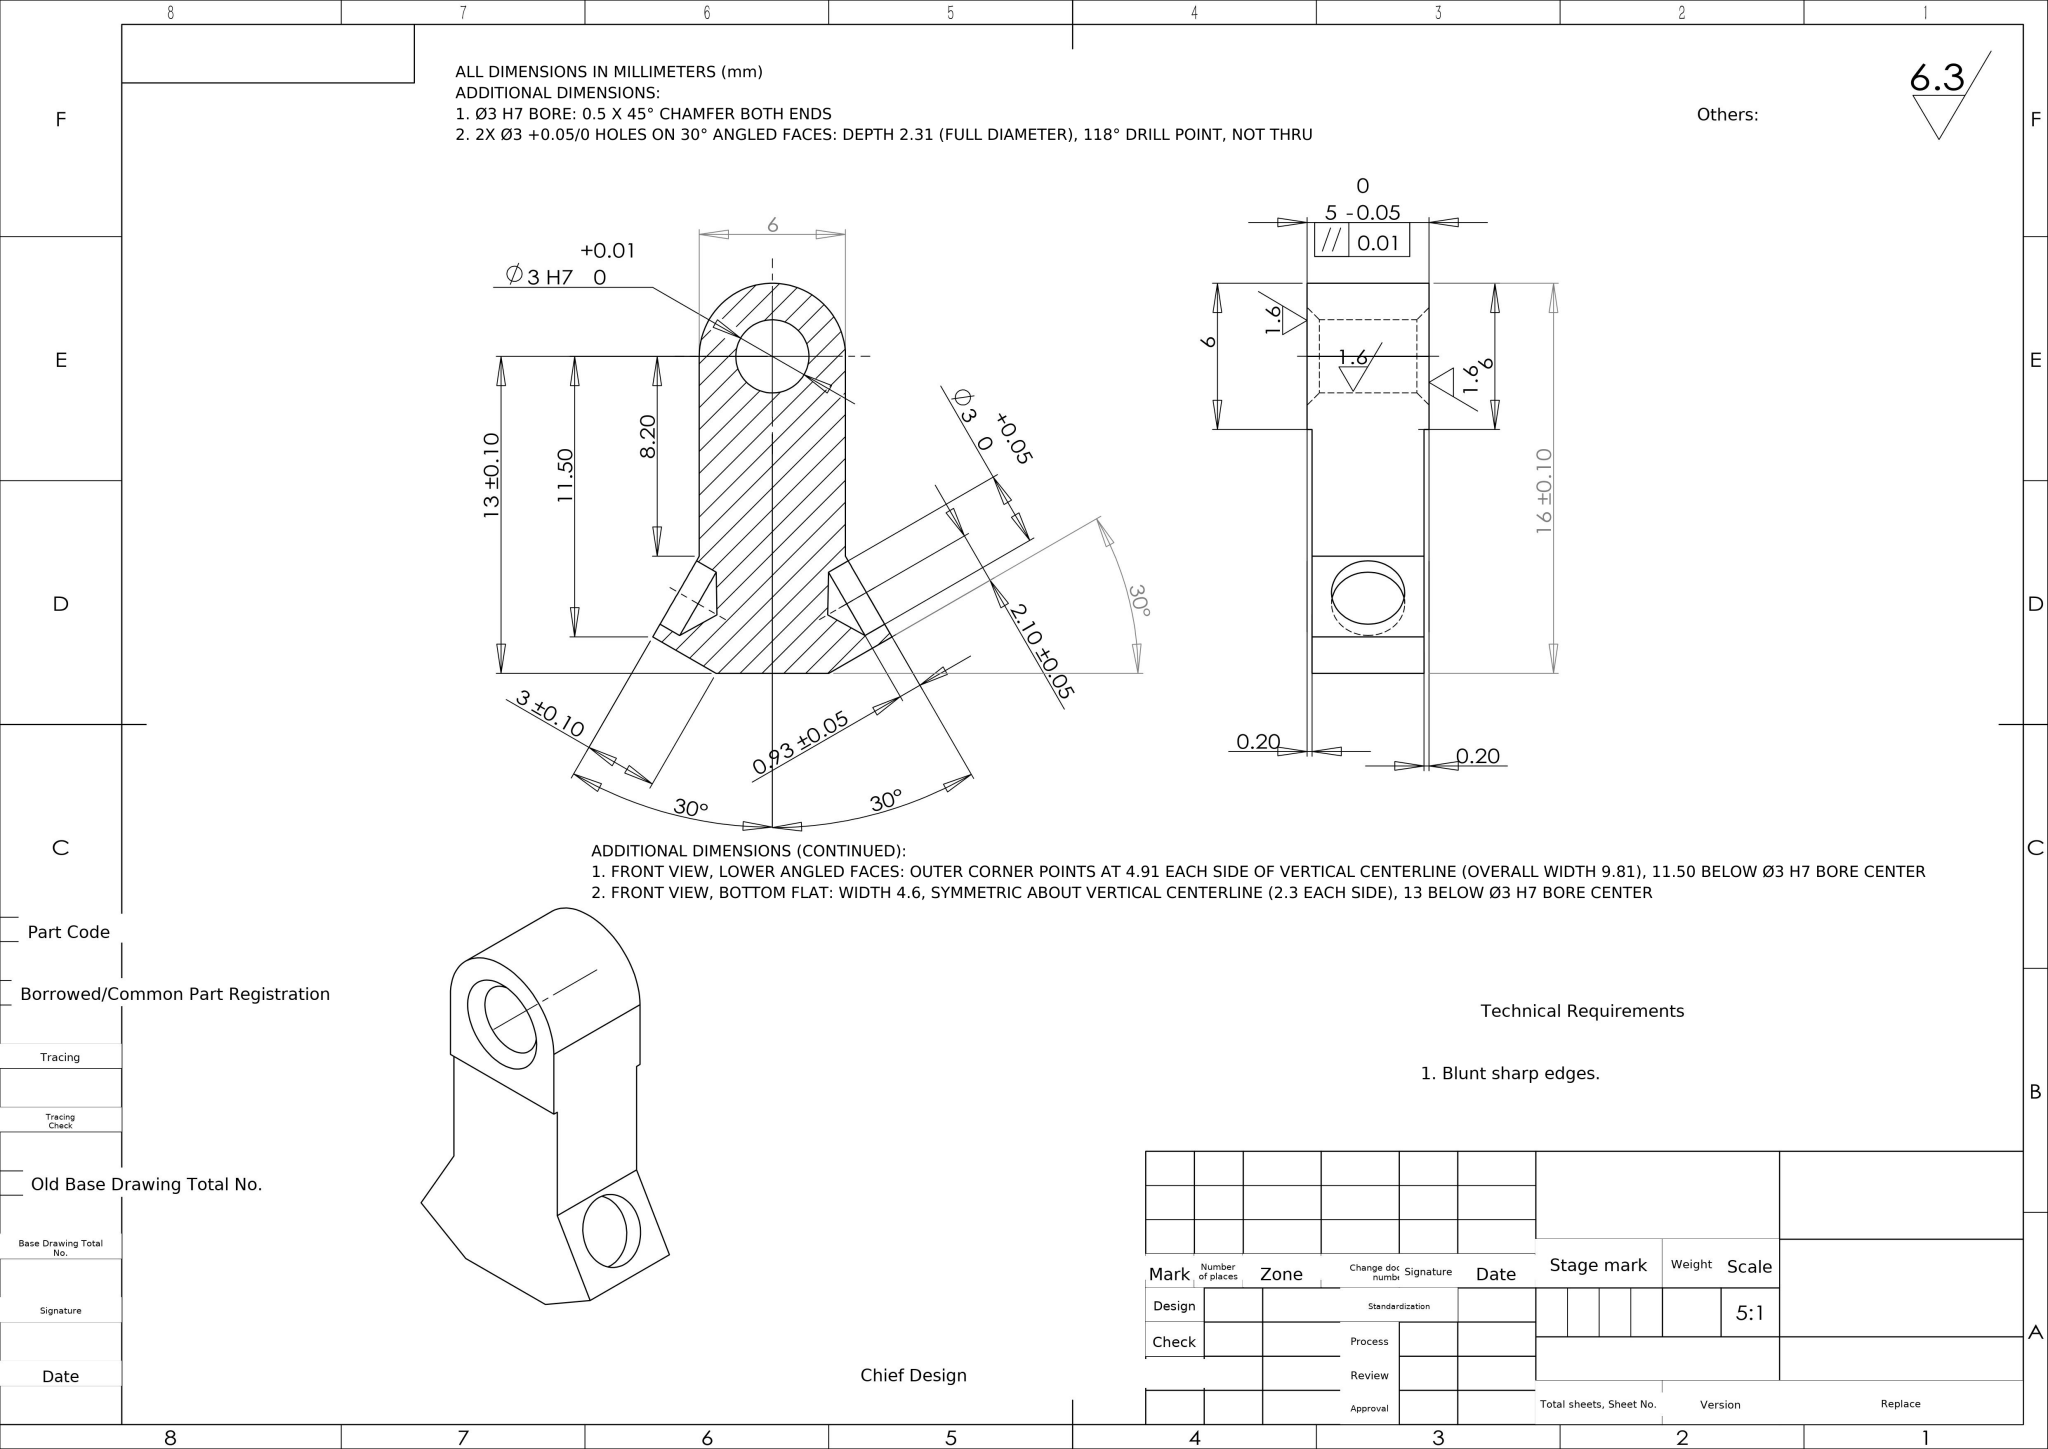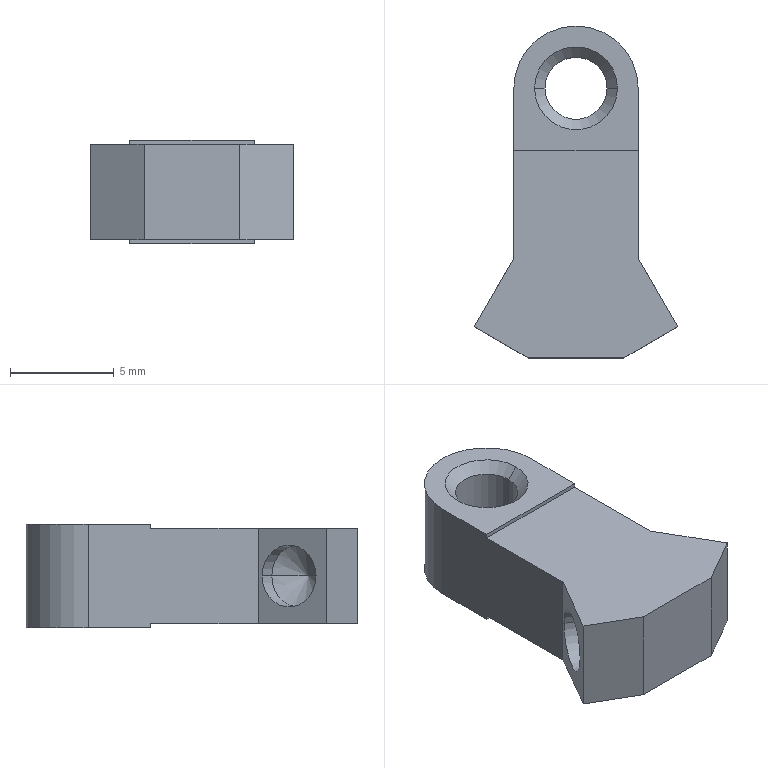Part | NX | mm | 1 solid | 28 faces | box 9.81 x 16 x 5 mm | volume 419 mm3 | plane 13 | cone 8 | cylinder 7 | commonest cylinder face diameters 3 x6 6 x1